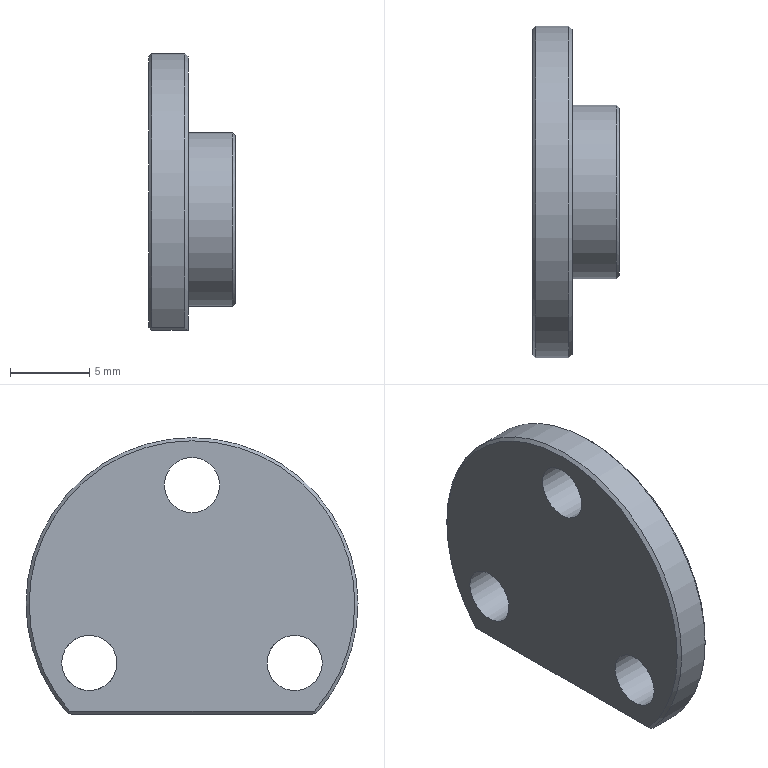Component | NX | DJZ_09_END_CAP | 1 solid | 18 faces | volume 949 mm3 | plane 8 | cylinder 6 | cone 4 | commonest cylinder face diameters 3.5 x3 21 x1 11 x1 3.1 x1